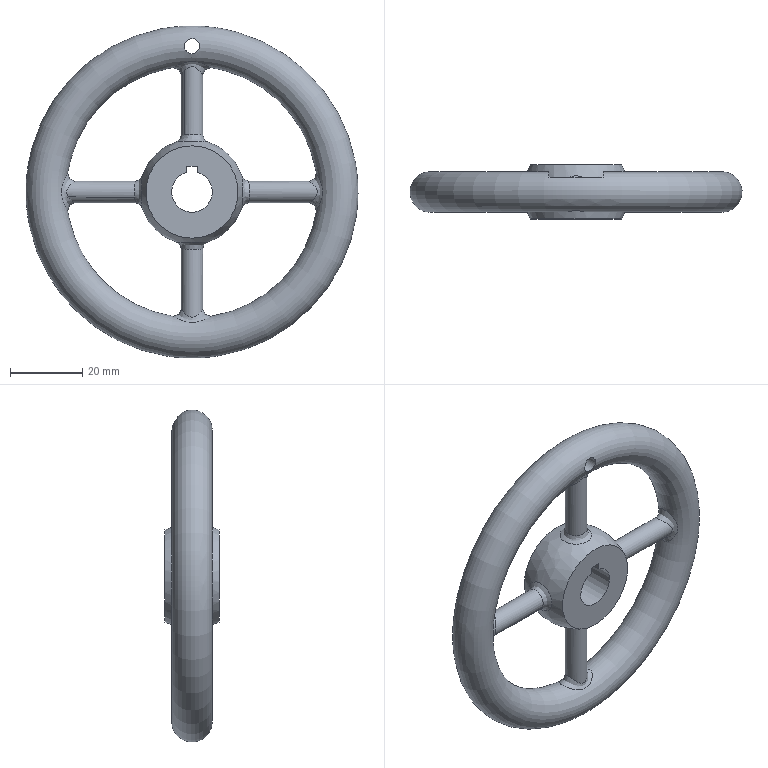Component | NX | TURNTABLE | 1 solid | 24 faces | volume 34886 mm3 | spline 9 | plane 8 | cylinder 6 | torus 1 | commonest cylinder face diameters 6 x4 11.3 x1 4.2 x1